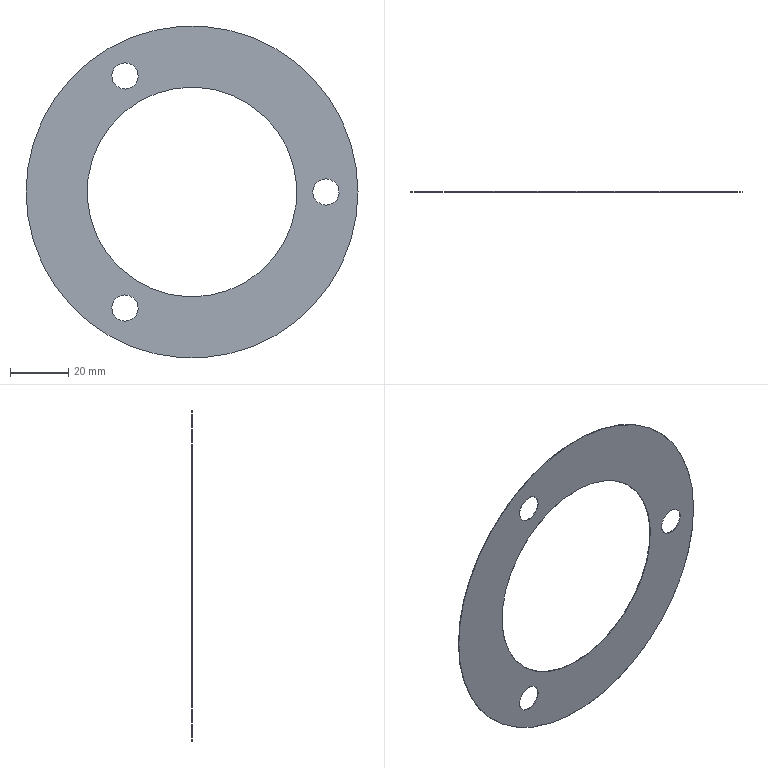Component | SolidWorks | 10-1 | 1 solid | 12 faces | box 114 x 0.2 x 114 mm | volume 1189 mm3 | cylinder 10 | plane 2 | commonest cylinder face diameters 9 x6 72 x2 114 x2
build123d program:
from build123d import *

# Parameters (mm, degrees)
SKETCH1_R           = 57
SKETCH1_R_2         = 36
SKETCH1_R_3         = 4.5
BOSS_EXTRUDE1_DEPTH = 0.2


with BuildPart() as part:
    # Sketch1 → Boss-Extrude1 (new body)
    with BuildSketch(Plane(origin=(0, 0, 0), x_dir=(1, 0, 0), z_dir=(0, 1, 0))):
        with Locations(Location((0, 0, 0), (0, 0, 270))):
            Circle(SKETCH1_R)
        with Locations(Location((0, 0, 0), (0, 0, 270))):
            Circle(SKETCH1_R_2, mode=Mode.SUBTRACT)
        with Locations(Location((0, -46, 0), (0, 0, 270))):
            Circle(SKETCH1_R_3, mode=Mode.SUBTRACT)
        with Locations(Location((-39.837, 23, 0), (0, 0, 270))):
            Circle(SKETCH1_R_3, mode=Mode.SUBTRACT)
        with Locations(Location((39.837, 23, 0), (0, 0, 270))):
            Circle(SKETCH1_R_3, mode=Mode.SUBTRACT)
    extrude(amount=BOSS_EXTRUDE1_DEPTH)


solid = part.part

# Placed as in the assembly
solid = solid.moved(Location((0, -288.2, 0), (0, 90, 0)))